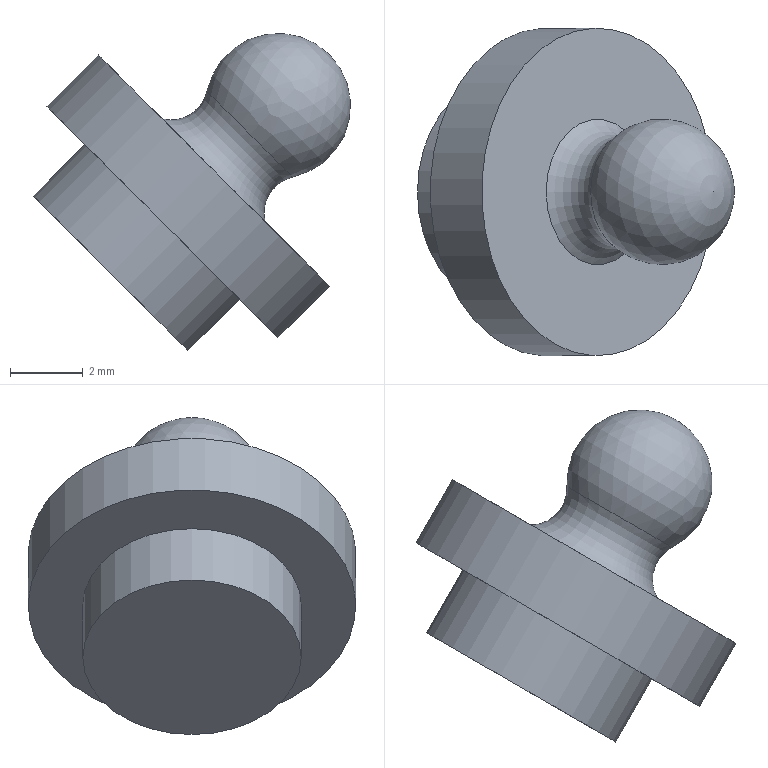Component | NX | VENT_END_CAP | 1 solid | 7 faces | volume 225 mm3 | plane 3 | cylinder 2 | sphere 1 | torus 1 | commonest cylinder face diameters 6 x1 9 x1